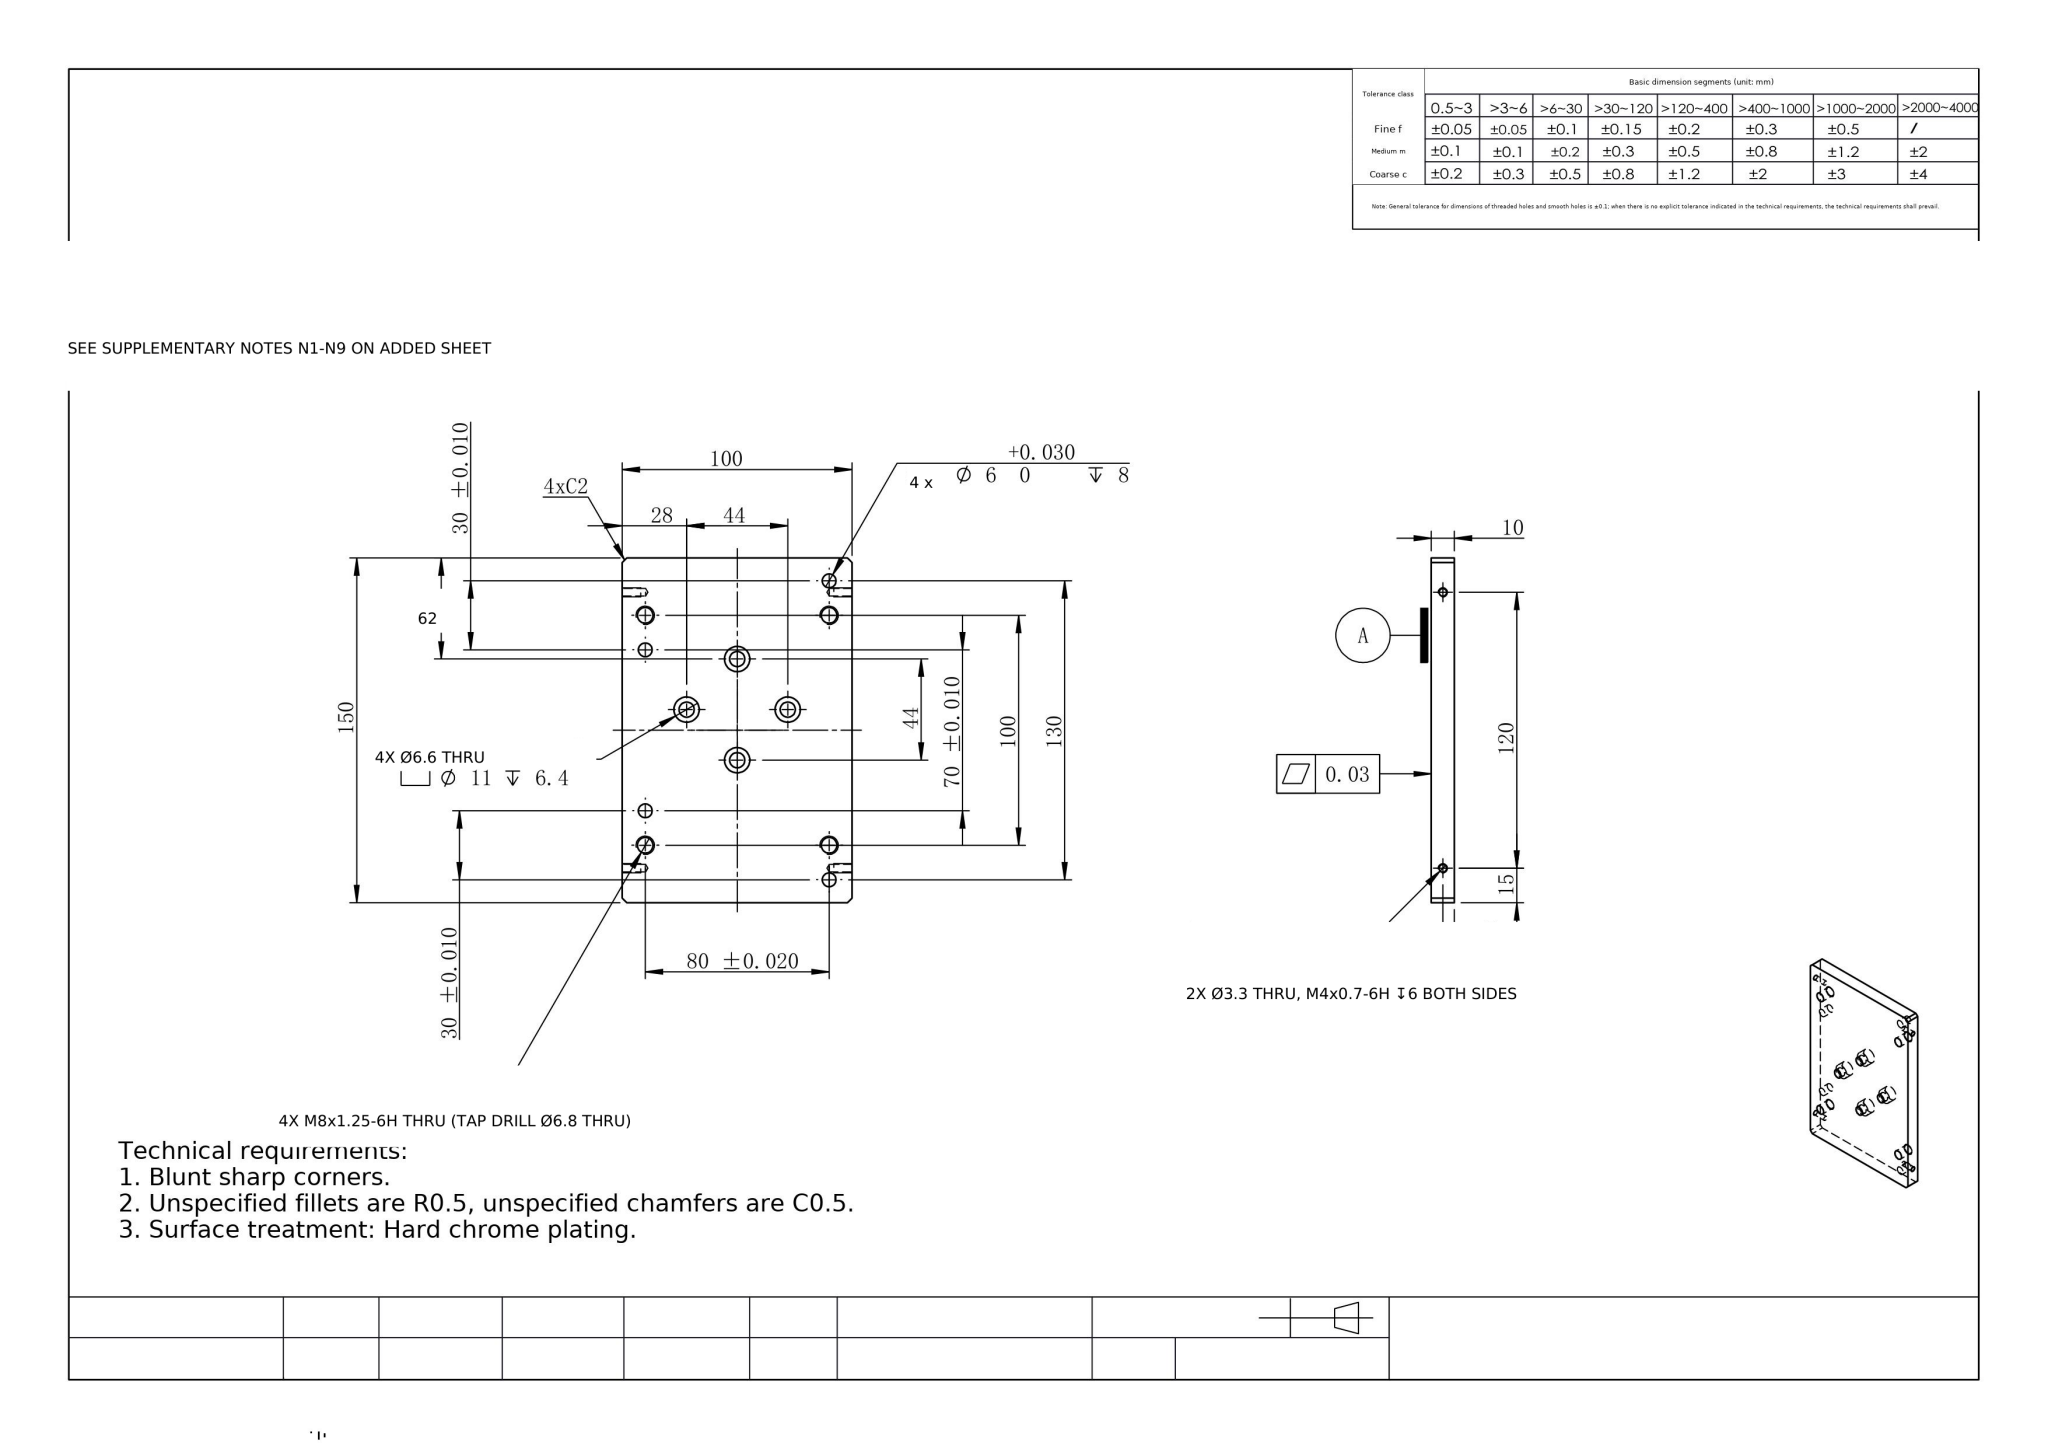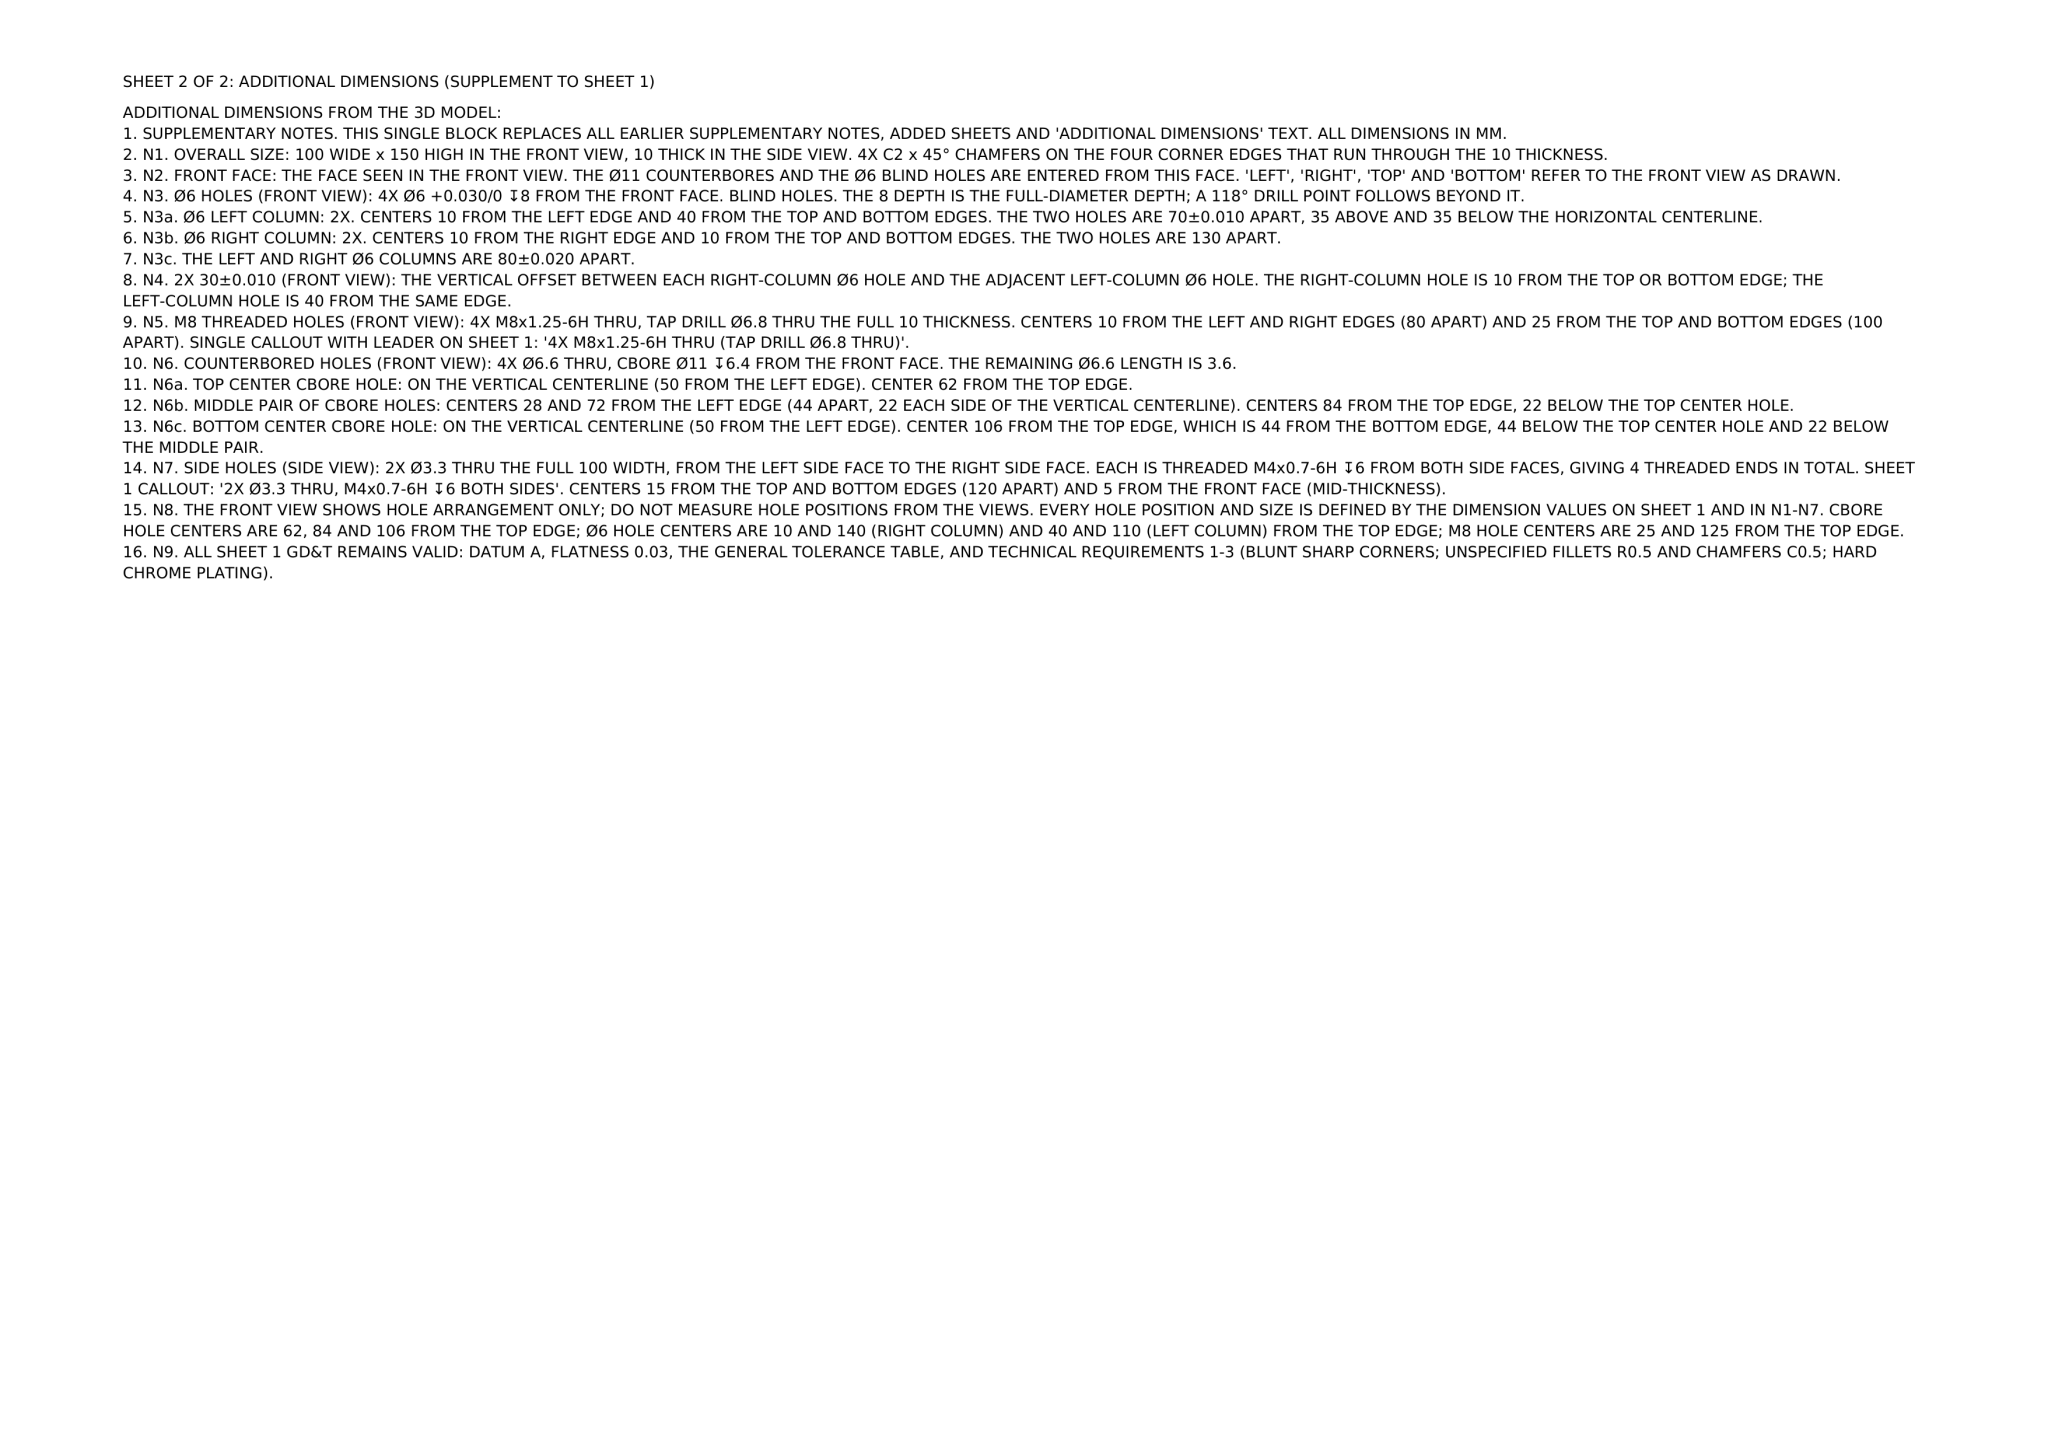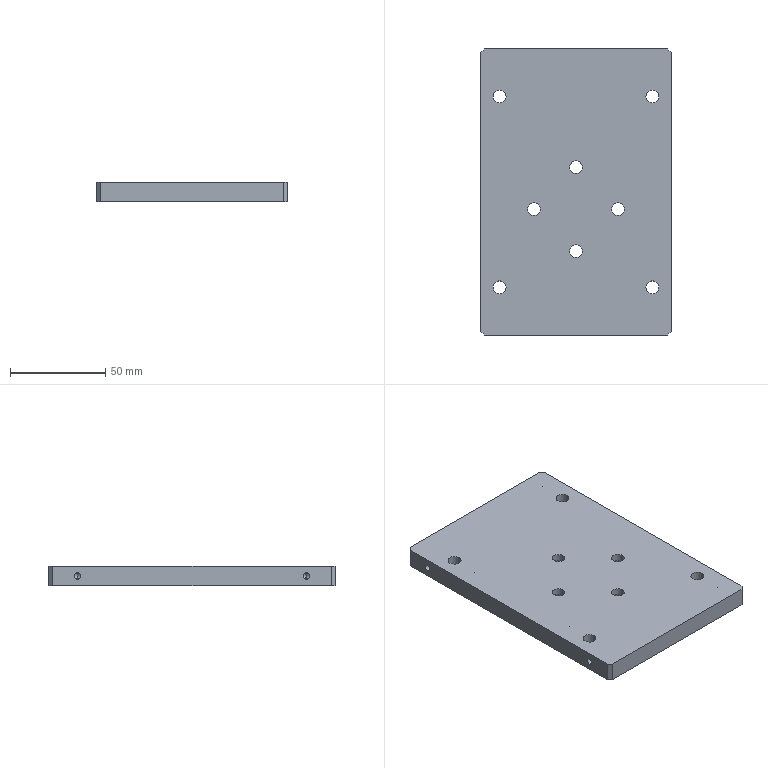Part | NX | mm | 1 solid | 70 faces | box 100 x 150 x 10 mm | volume 144214 mm3 | cylinder 40 | cone 16 | plane 14 | commonest cylinder face diameters 3.3 x8 11 x8 6.6 x8 6 x8 6.8 x8